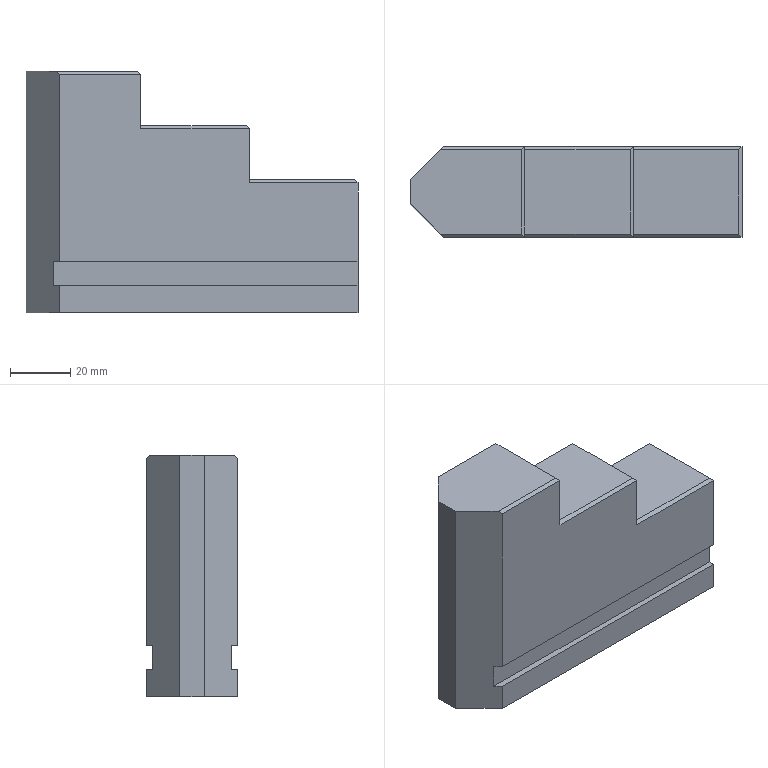Component | NX | JAW_2 | 1 solid | 29 faces | volume 192658 mm3 | plane 29